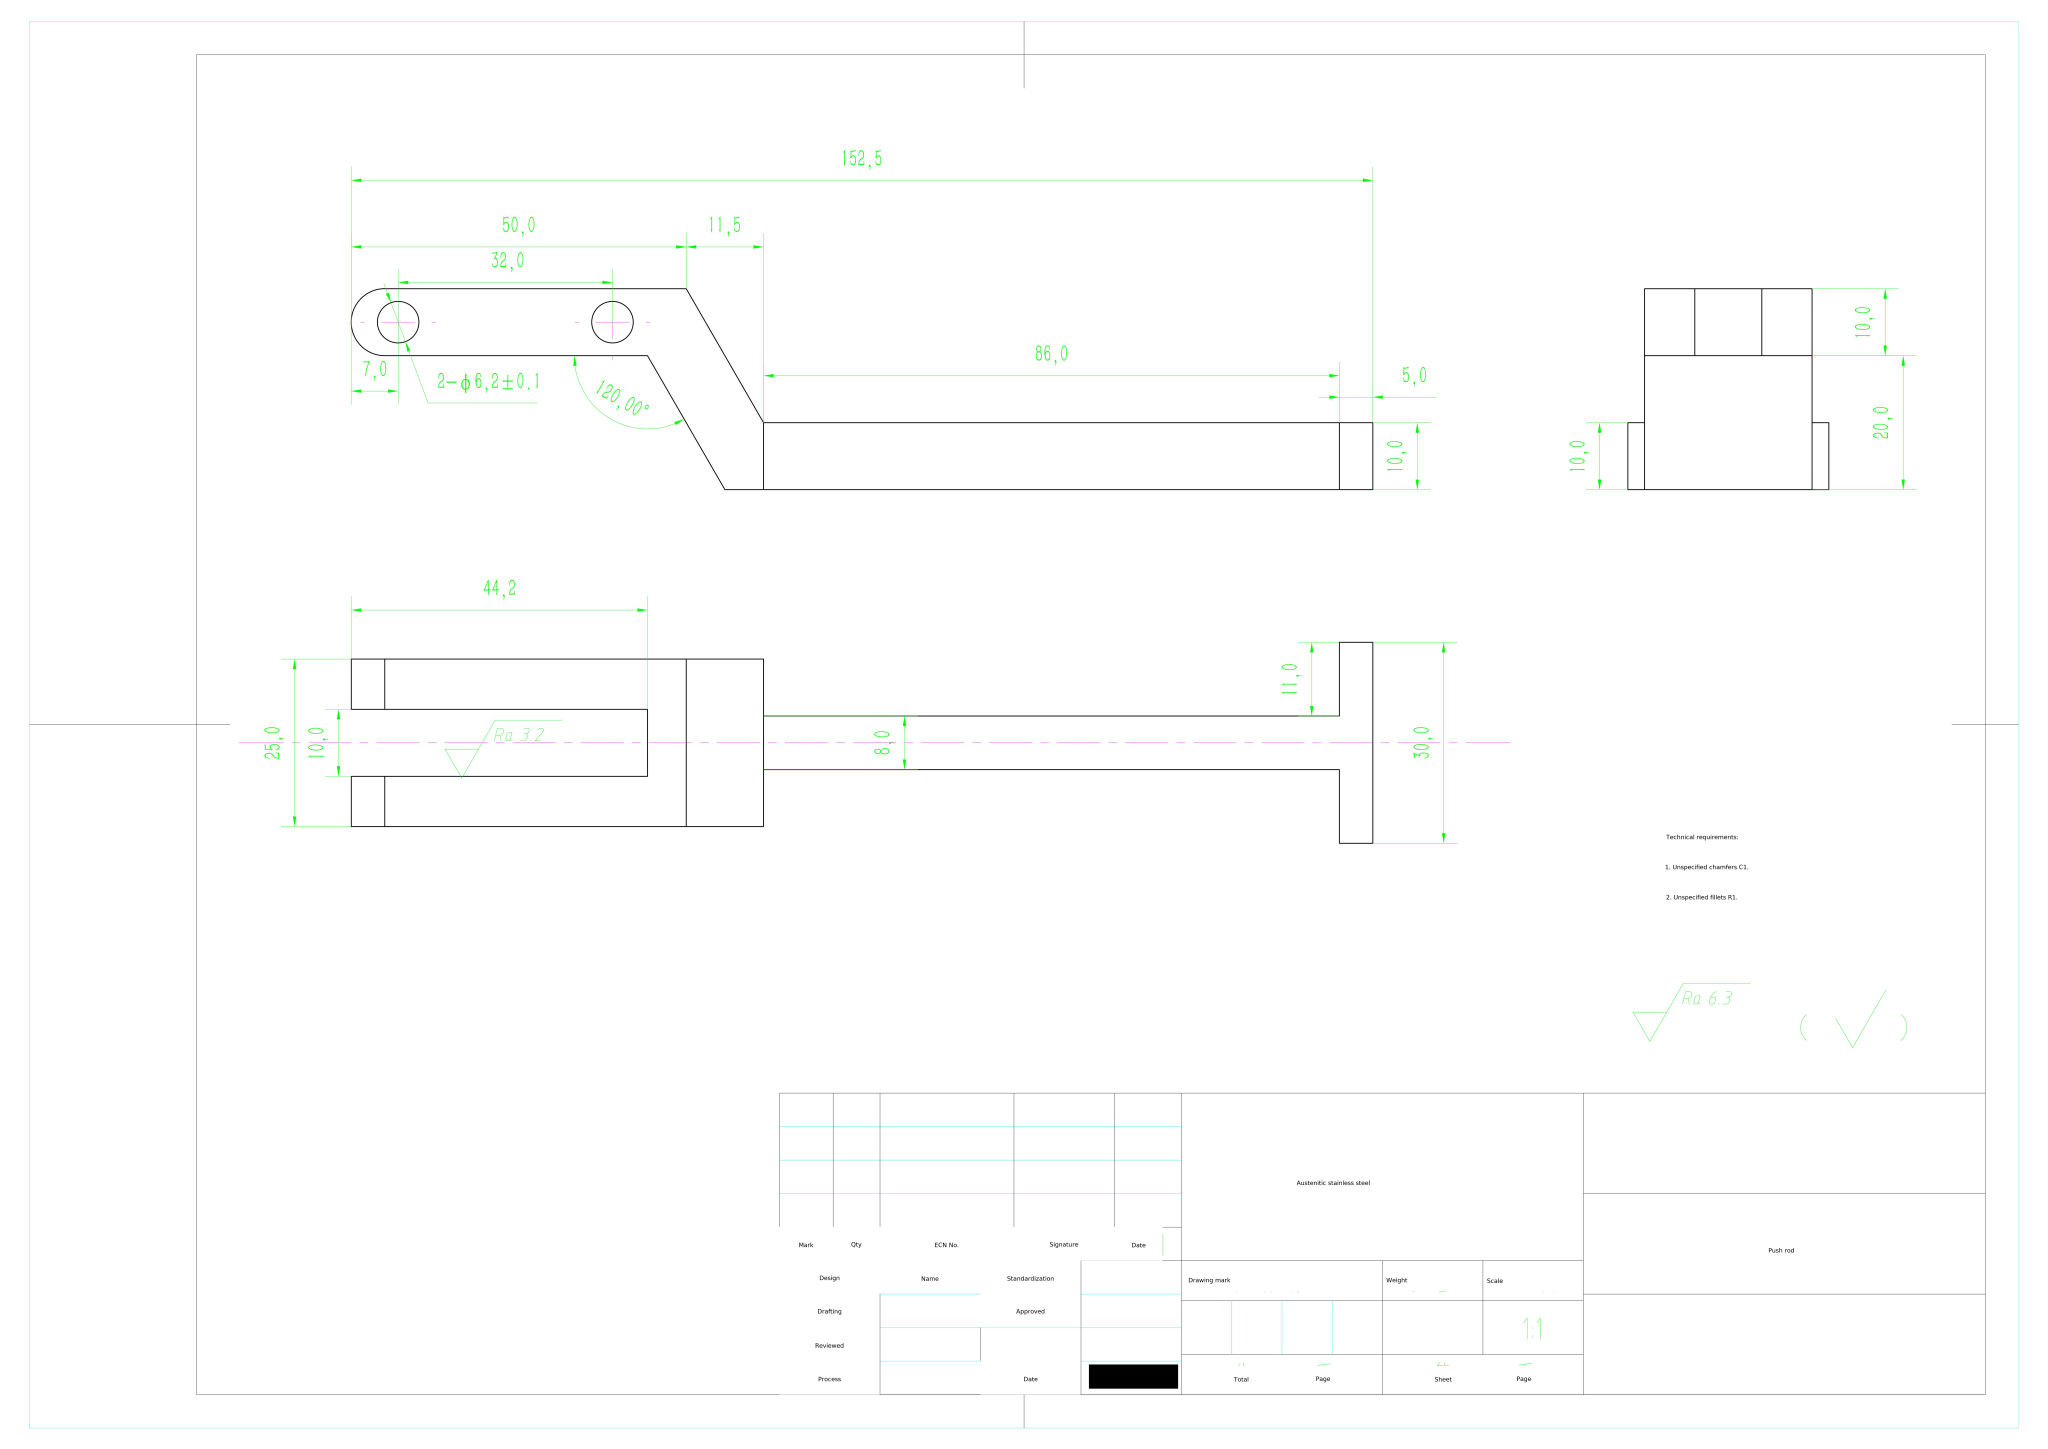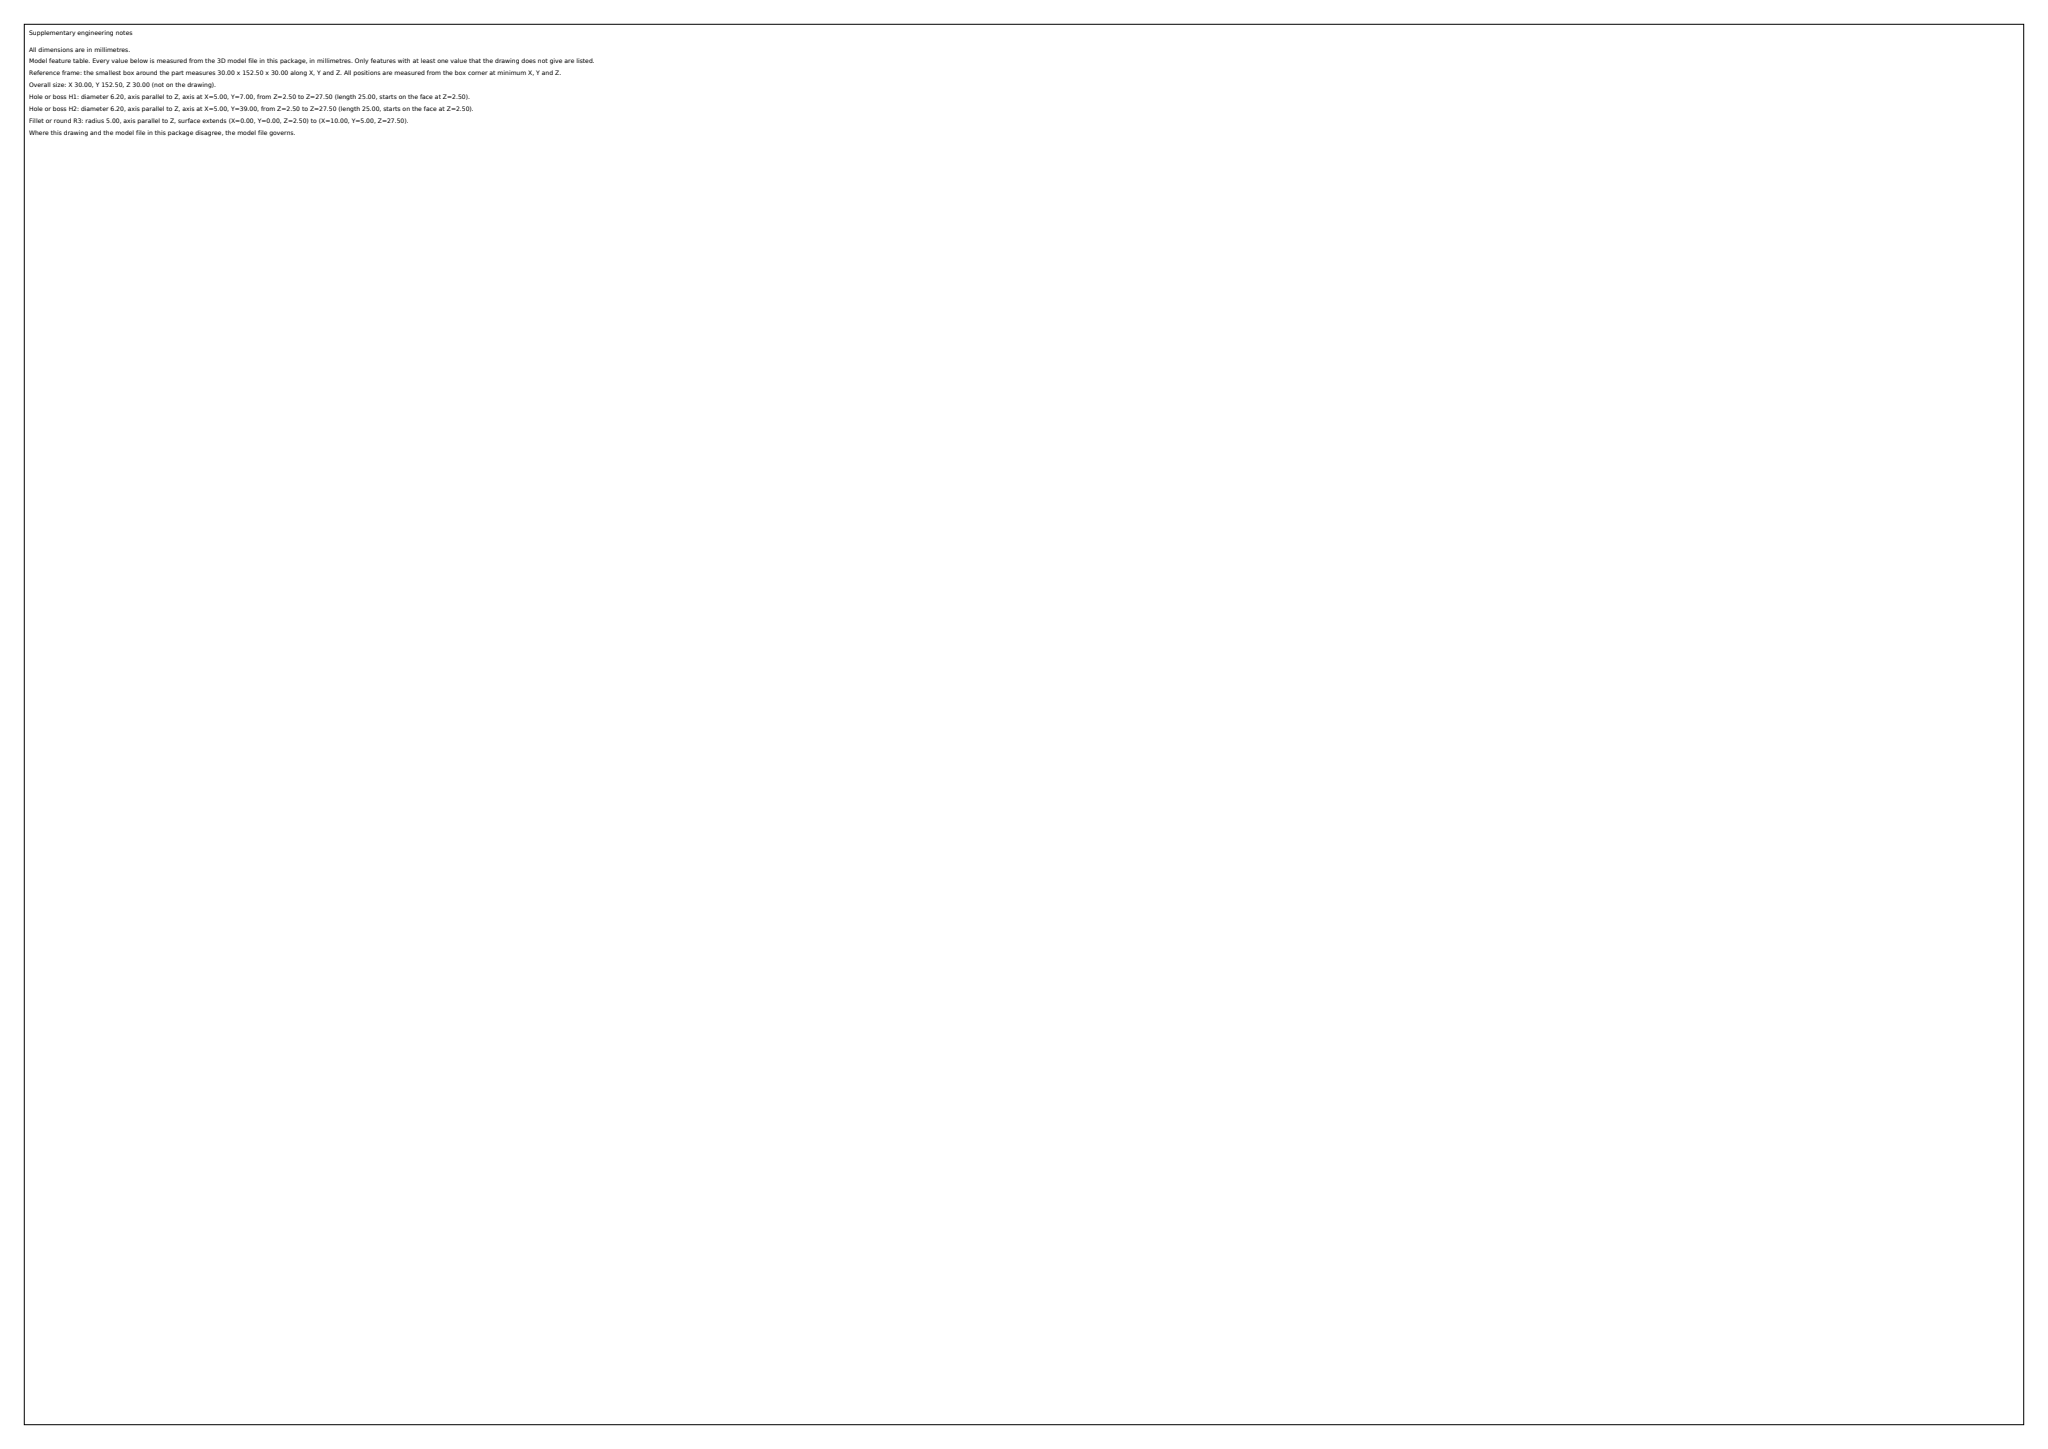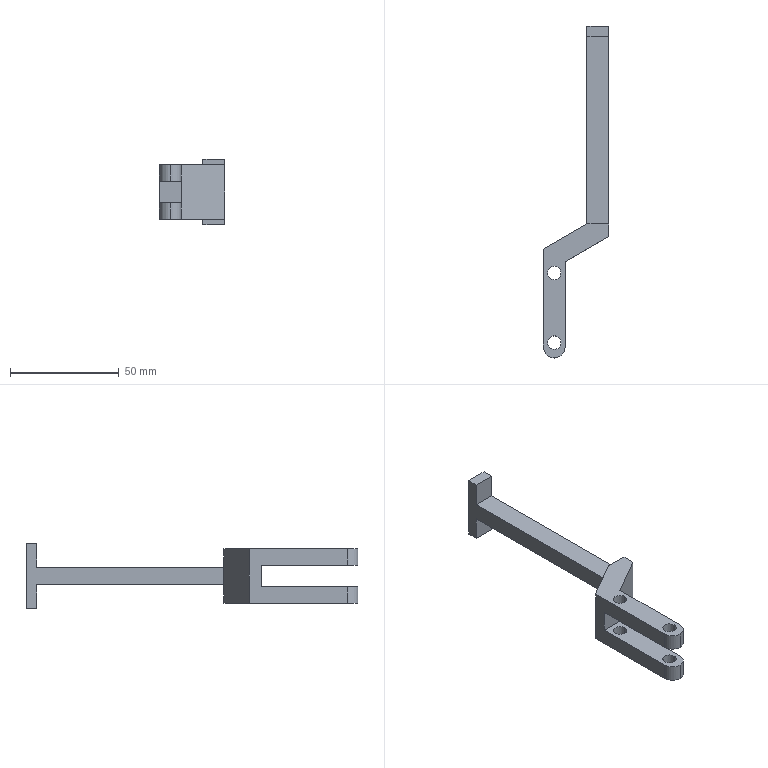Part | SolidWorks | mm | material Austenitic stainless steel | 1 solid | 33 faces | box 30 x 152.5 x 30 mm | volume 21160 mm3 | plane 21 | cylinder 12 | commonest cylinder face diameters 6.2 x8 10 x4